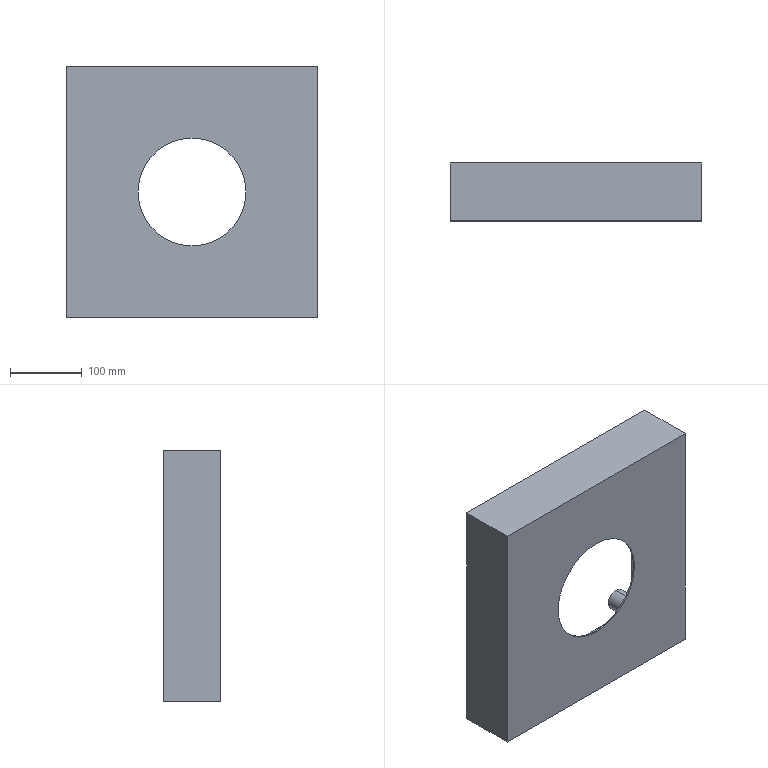Component | SolidWorks | InsectTrapLamp-1_InsectTrapLampBase-1 | 1 solid | 63 faces | volume 4579881 mm3 | cylinder 32 | plane 27 | spline 4 | commonest cylinder face diameters 5 x16 15 x8 30 x6 150 x2